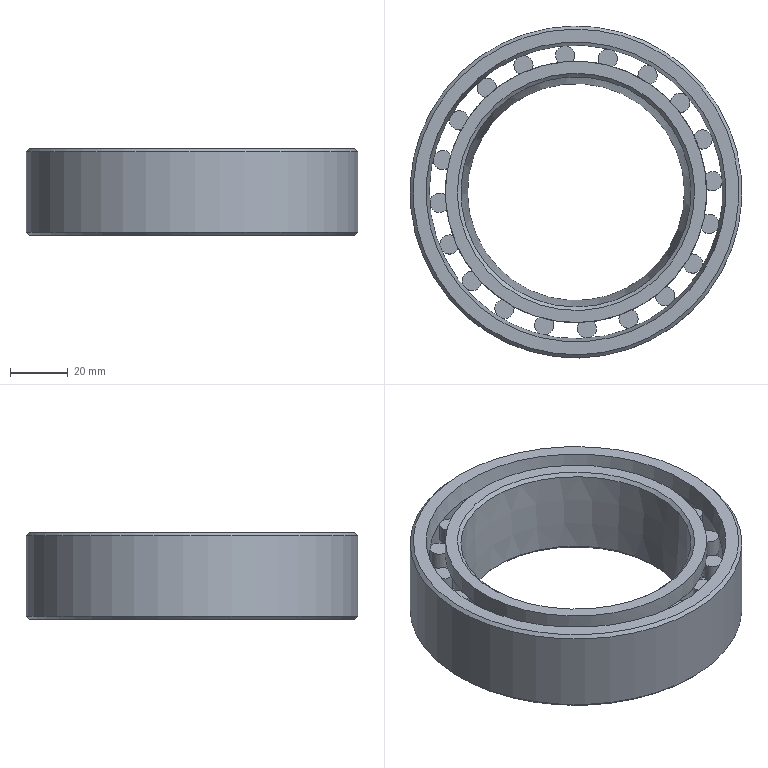Component | NX | CA6140-ZHUZHOU-E3182115 | 42 solids | 142 faces | volume 121219 mm3 | plane 88 | cylinder 47 | cone 7 | commonest cylinder face diameters 6.667 x40 90.533 x3 88.3 x2 115 x1 101.7 x1